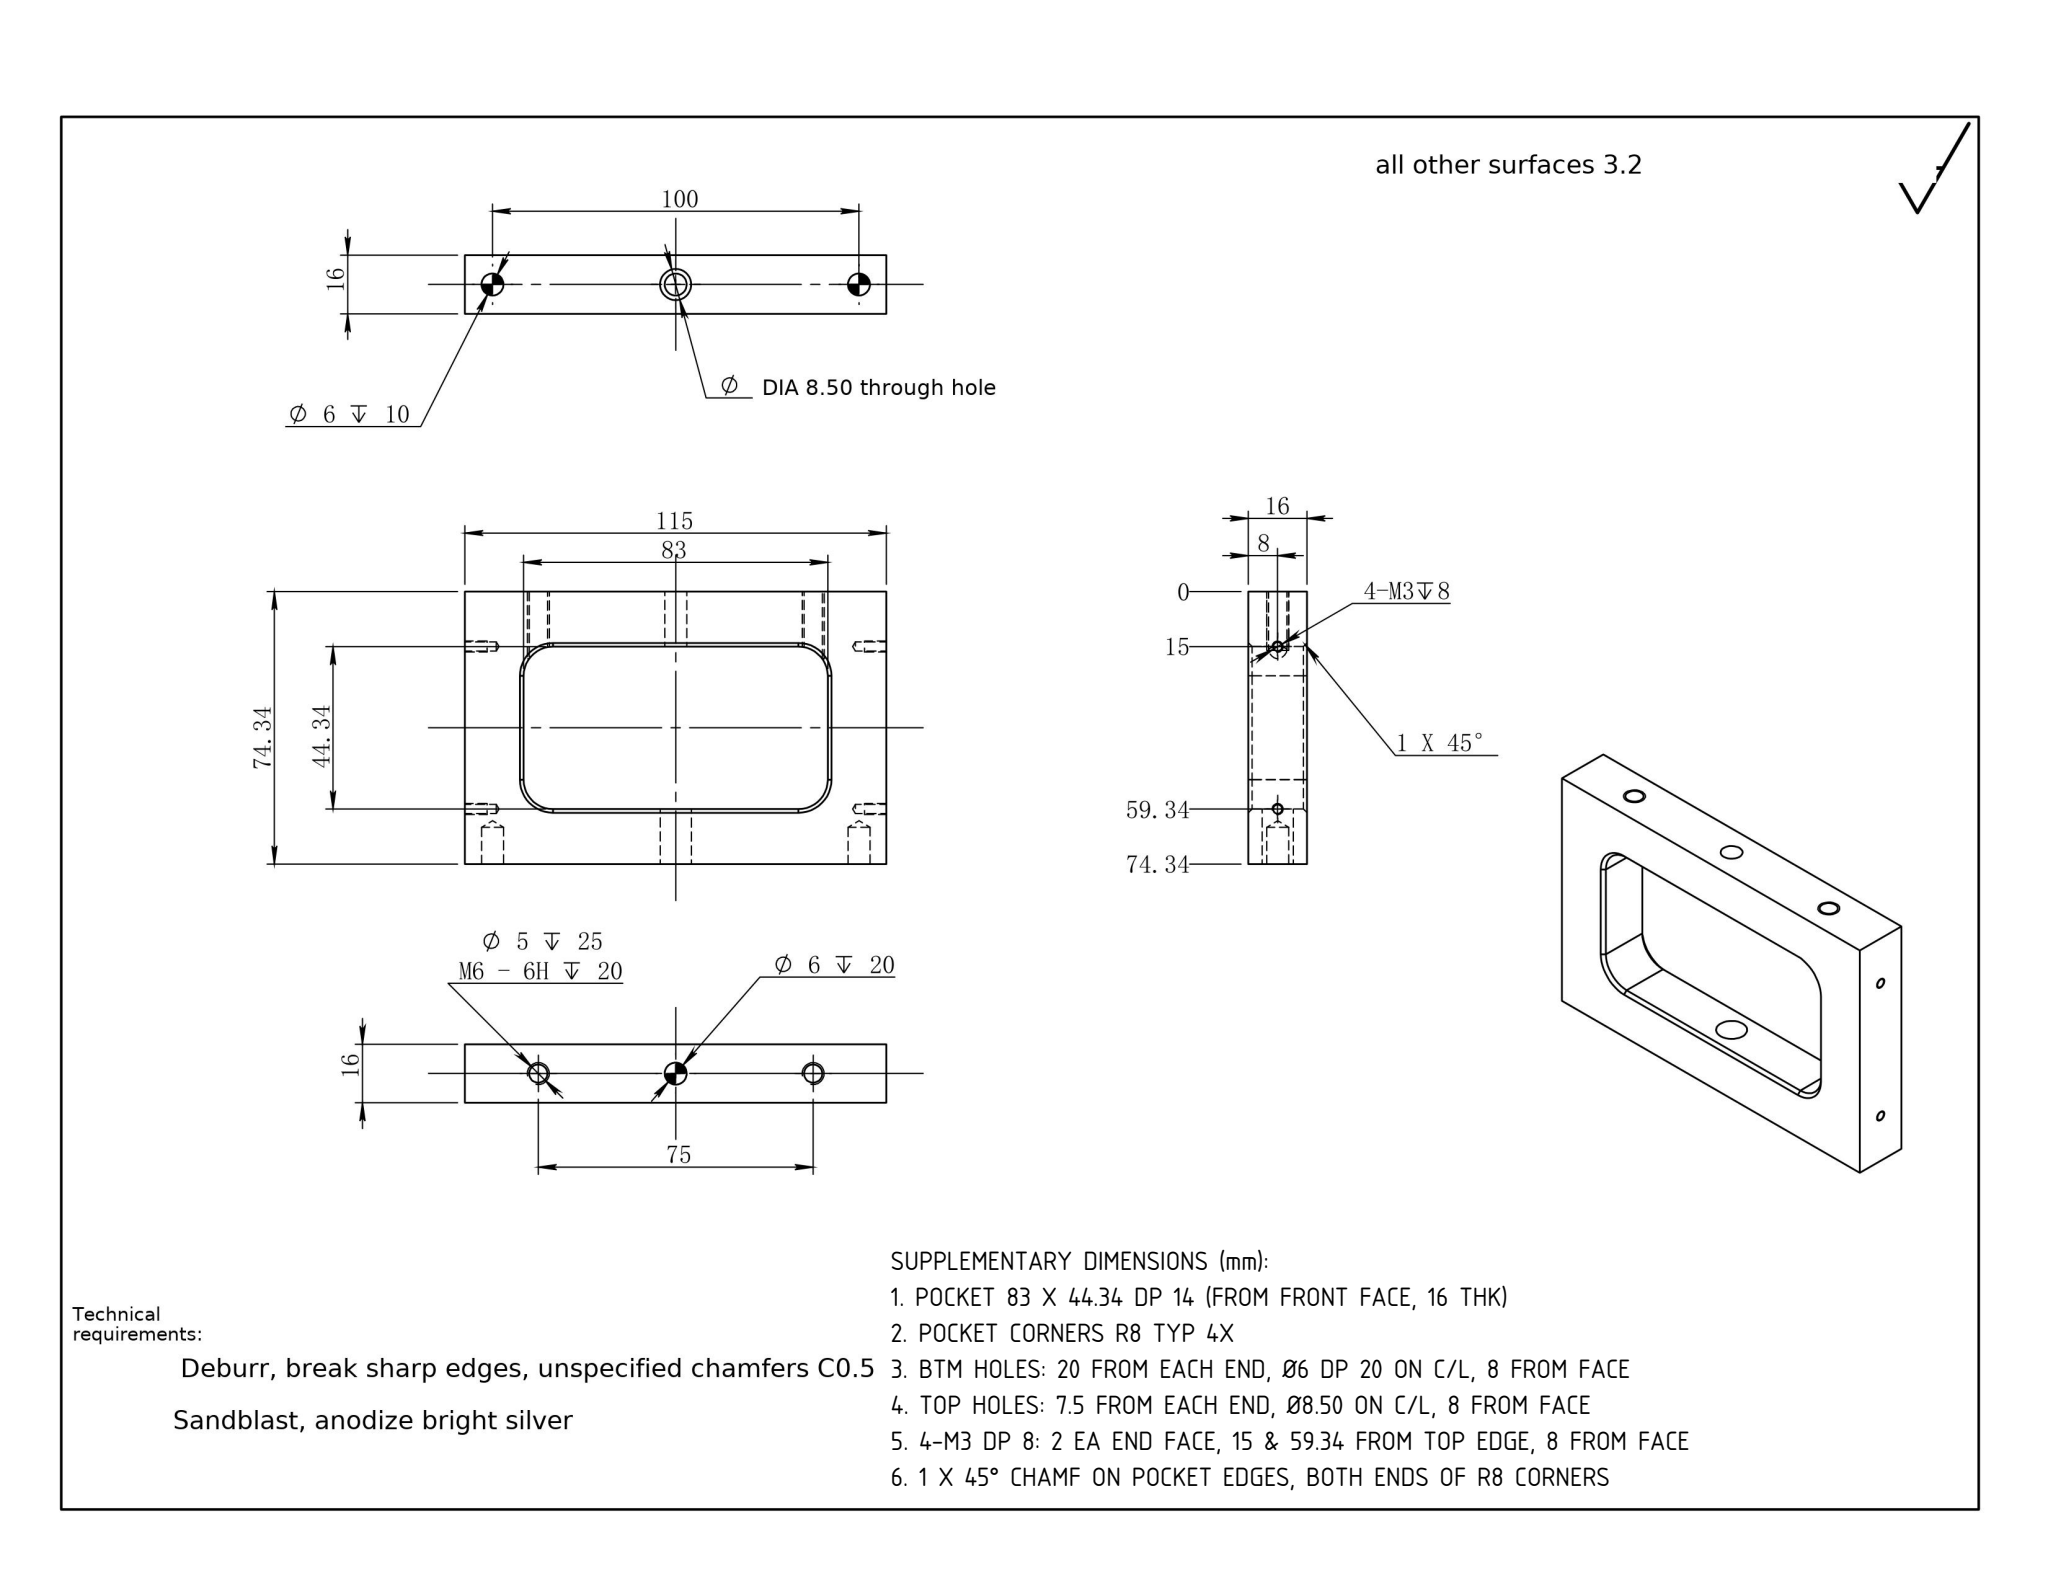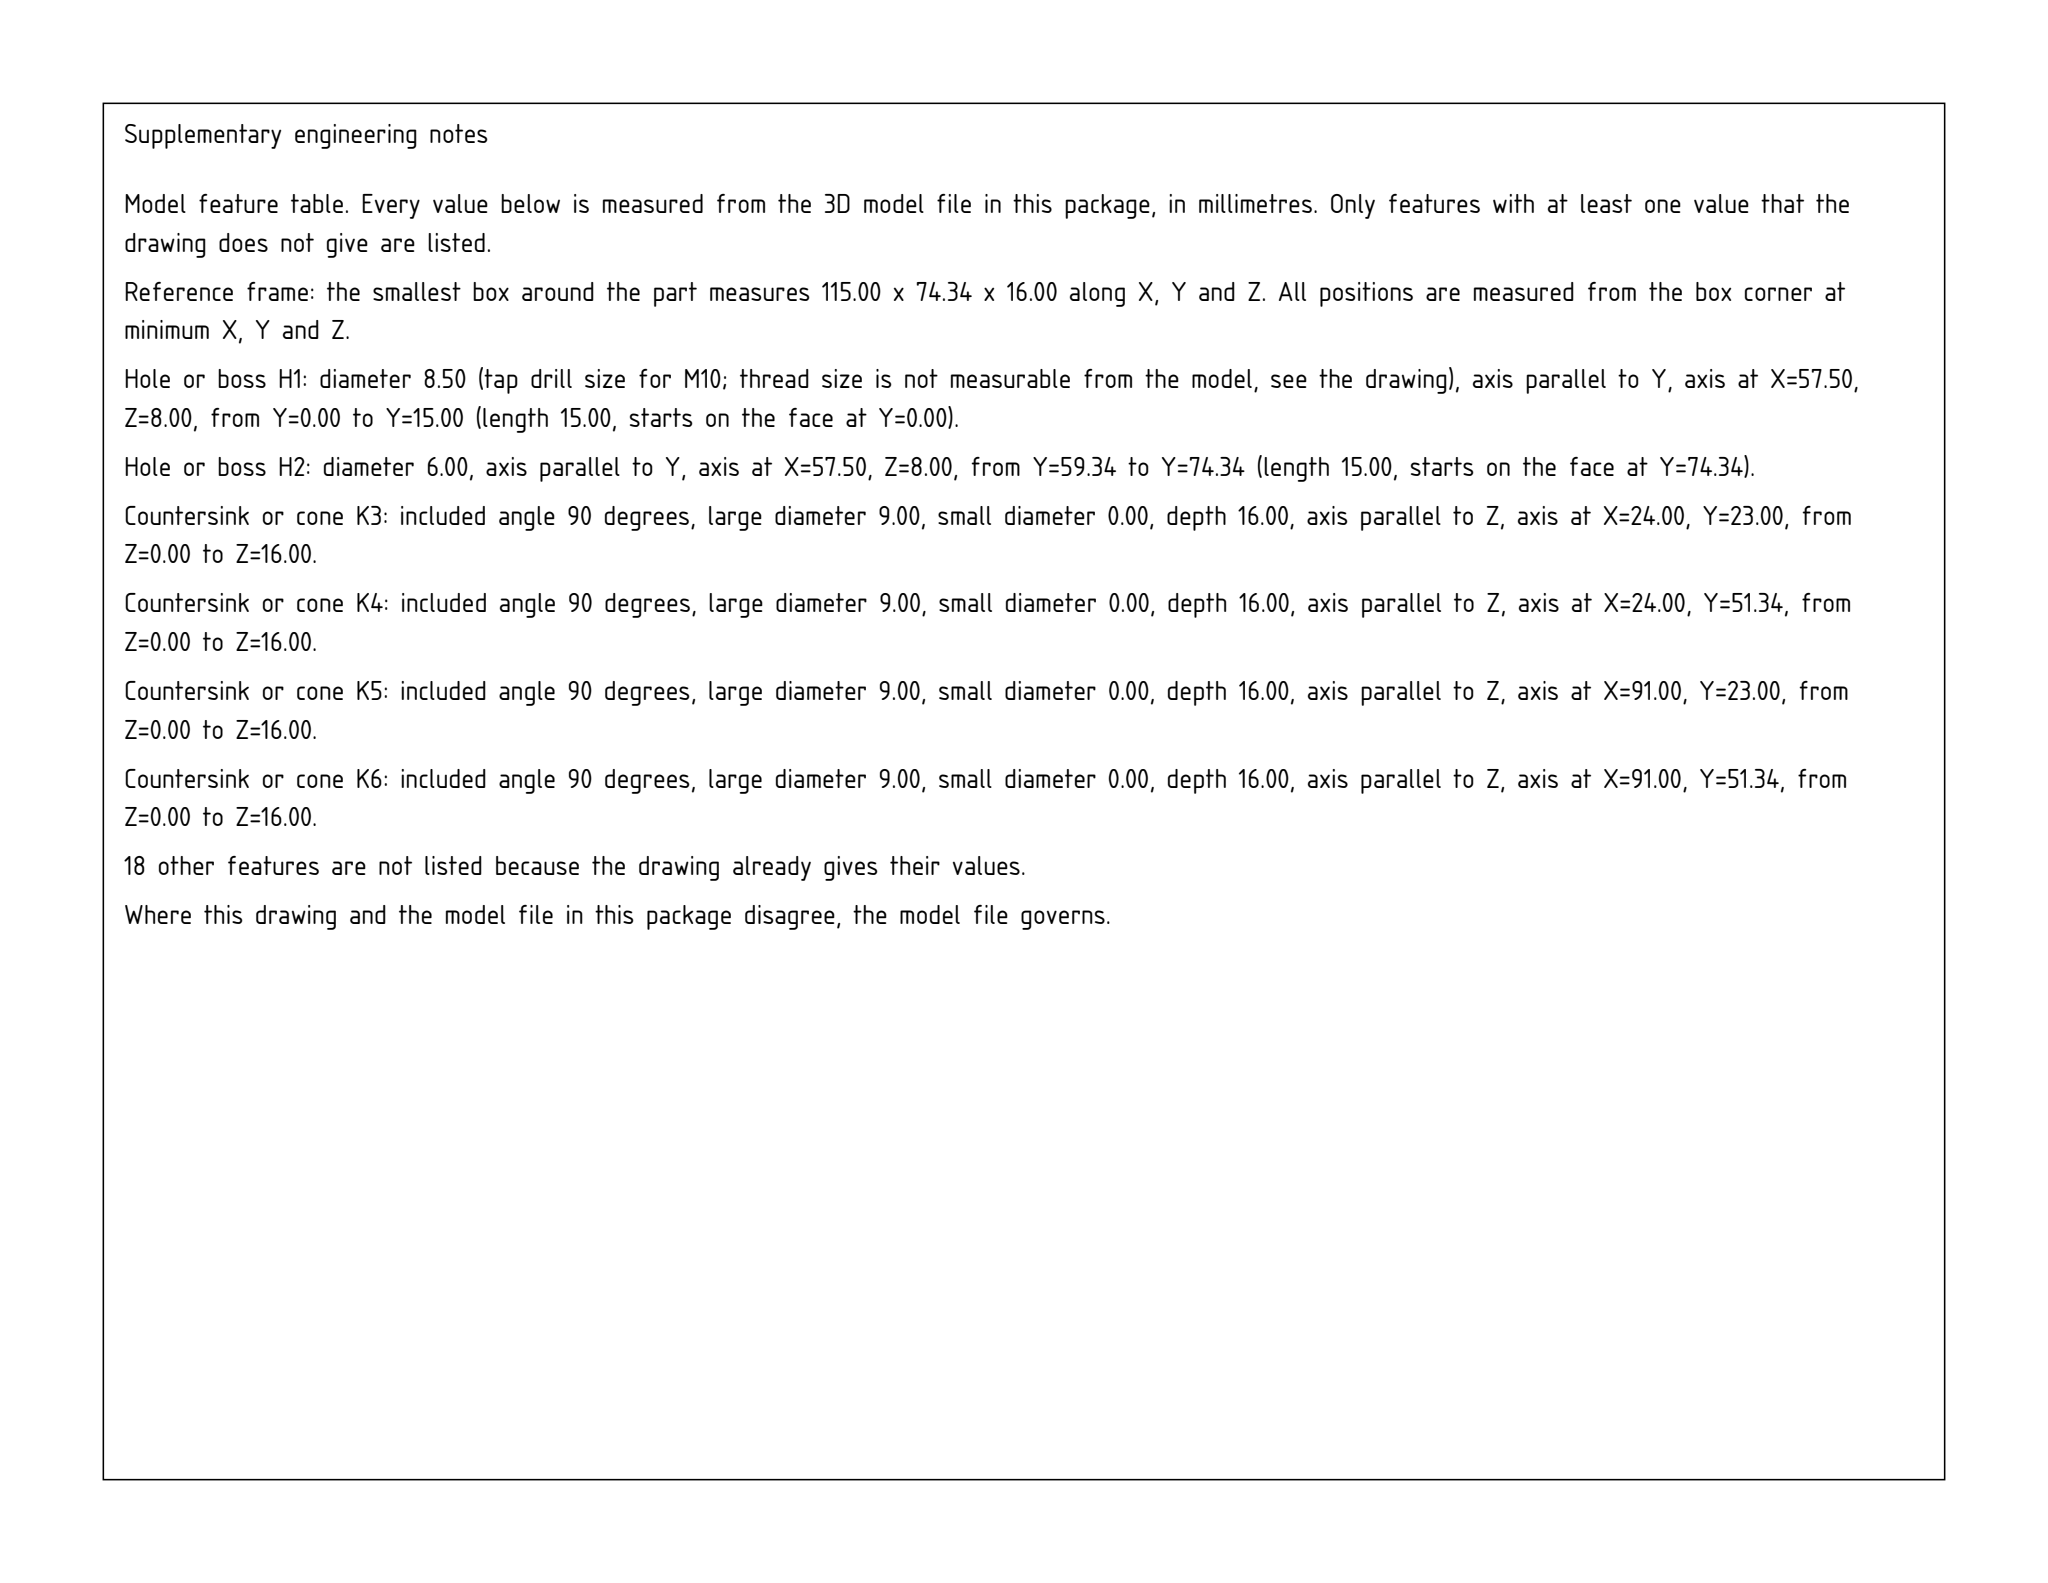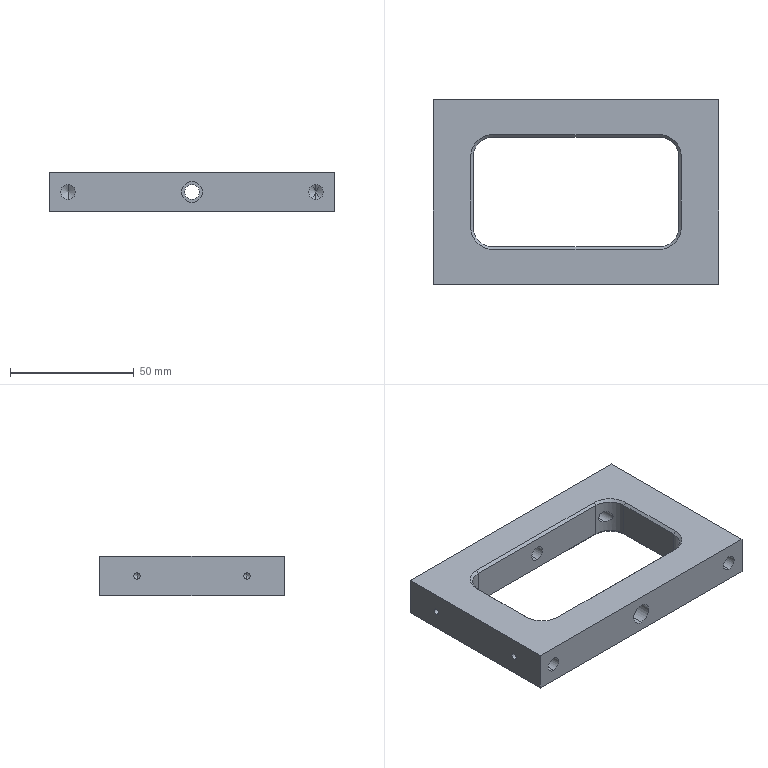Part | SolidWorks | mm | 1 solid | 62 faces | box 115 x 74.34 x 16 mm | volume 75854 mm3 | cylinder 24 | cone 20 | plane 18 | commonest cylinder face diameters 2.5 x8 6 x6 5 x4 16 x4 8.5 x2
build123d program:
from build123d import *

# Parameters (mm, degrees)
SKETCH1_W                      = 115
SKETCH1_H                      = 16
BOSS_EXTRUDE1_DEPTH            = 74.34
SKETCH11_W                     = 83
SKETCH11_H                     = 44.34
CUT_EXTRUDE1_DEPTH             = 96.335
FILLET1_R                      = 8
F_6_0_6_DIAMETER_HOLE2_D       = 6
F_6_0_6_DIAMETER_HOLE2_DEPTH   = 10
F_6_0_6_DIAMETER_HOLE2_TIP     = 1.803
F_6_0_6_DIAMETER_HOLE1_D       = 6
F_6_0_6_DIAMETER_HOLE1_DEPTH   = 20
F_6_0_6_DIAMETER_HOLE1_TIP     = 1.803
M6_TAPPED_HOLE2_D              = 5
M6_TAPPED_HOLE2_DEPTH          = 25
M6_TAPPED_HOLE2_TIP            = 1.502
F_8_5_8_5_DIAMETER_HOLE1_D     = 8.5
F_8_5_8_5_DIAMETER_HOLE1_DEPTH = 15
CHAMFER1_SIZE                  = 1
M3_TAPPED_HOLE1_AT_2_COUNT     = 2
M3_TAPPED_HOLE1_AT_2_PITCH     = 44.34


with BuildPart() as part:
    # Sketch1 → Boss-Extrude1 (new body)
    with BuildSketch(Plane(origin=(0, 0, 0), x_dir=(1, 0, 0), z_dir=(0, 1, 0))):
        Rectangle(SKETCH1_W, SKETCH1_H)
    extrude(amount=BOSS_EXTRUDE1_DEPTH)

    # Sketch11 → Cut-Extrude1 (cut, through all)
    with BuildSketch(Plane.XY.offset(8)):
        with Locations((0, 37.17)):
            Rectangle(SKETCH11_W, SKETCH11_H)
    extrude(amount=-CUT_EXTRUDE1_DEPTH, mode=Mode.SUBTRACT)

    # Fillet1
    fillet1_edges = [part.edges().sort_by_distance(p)[0] for p in [
        (41.5, 59.34, 0),
        (41.5, 15, 0),
        (-41.5, 15, 0),
        (-41.5, 59.34, 0),
    ]]
    fillet(fillet1_edges, radius=FILLET1_R)

    # 6.0 _6_ Diameter Hole2
    with Locations(Plane(origin=(0, 0, 0), x_dir=(-1, 0, 0), z_dir=(0, -1, 0))):
        with Locations((-50, 0), (50, 0)):
            Hole(F_6_0_6_DIAMETER_HOLE2_D / 2, depth=F_6_0_6_DIAMETER_HOLE2_DEPTH)
            with Locations((0, 0, -(F_6_0_6_DIAMETER_HOLE2_DEPTH + F_6_0_6_DIAMETER_HOLE2_TIP / 2))):  # 118° drill point
                Cone(0, F_6_0_6_DIAMETER_HOLE2_D / 2, F_6_0_6_DIAMETER_HOLE2_TIP, mode=Mode.SUBTRACT)

    # 6.0 _6_ Diameter Hole1
    with Locations(Plane(origin=(0, 74.34, 0), x_dir=(-1, 0, 0), z_dir=(0, 1, 0))):
        with Locations((0, 0)):
            Hole(F_6_0_6_DIAMETER_HOLE1_D / 2, depth=F_6_0_6_DIAMETER_HOLE1_DEPTH)
            with Locations((0, 0, -(F_6_0_6_DIAMETER_HOLE1_DEPTH + F_6_0_6_DIAMETER_HOLE1_TIP / 2))):  # 118° drill point
                Cone(0, F_6_0_6_DIAMETER_HOLE1_D / 2, F_6_0_6_DIAMETER_HOLE1_TIP, mode=Mode.SUBTRACT)

    # M6 Tapped Hole2
    with Locations(Plane(origin=(0, 74.34, 0), x_dir=(1, 0, 0), z_dir=(0, 1, 0))):
        with Locations((-37.5, 0), (37.5, 0)):
            Hole(M6_TAPPED_HOLE2_D / 2, depth=M6_TAPPED_HOLE2_DEPTH)
            with Locations((0, 0, -(M6_TAPPED_HOLE2_DEPTH + M6_TAPPED_HOLE2_TIP / 2))):  # 118° drill point
                Cone(0, M6_TAPPED_HOLE2_D / 2, M6_TAPPED_HOLE2_TIP, mode=Mode.SUBTRACT)

    # 8.5 _8.5_ Diameter Hole1
    with Locations(Plane(origin=(0, 15, 0), x_dir=(1, 0, 0), z_dir=(0, 1, 0))):
        with Locations((0, 0)):
            Hole(F_8_5_8_5_DIAMETER_HOLE1_D / 2, depth=F_8_5_8_5_DIAMETER_HOLE1_DEPTH)

    # Chamfer1
    chamfer1_edges = [part.edges().sort_by_distance(p)[0] for p in [
        (41.5, 37.17, 8),
        (41.5, 37.17, -8),
        (0, 15, 8),
        (0, 15, -8),
        (0, 59.34, 8),
        (0, 59.34, -8),
        (-41.5, 37.17, 8),
        (-41.5, 37.17, -8),
        (39.157, 17.343, 8),
        (39.157, 17.343, -8),
        (39.157, 56.997, 8),
        (39.157, 56.997, -8),
        (-39.157, 56.997, 8),
        (-39.157, 56.997, -8),
        (-39.157, 17.343, 8),
        (-39.157, 17.343, -8),
    ]]
    chamfer(chamfer1_edges, length=CHAMFER1_SIZE)

    # Sketch15 → M3 Tapped Hole1 (revolve, cut)
    with BuildSketch(Plane(origin=(57.5, 59.34, 0), x_dir=(0, 0, -1), z_dir=(0, 1, 0))):
        Polygon((0, 0), (0, 9.251), (1.25, 8.5), (1.25, 0), align=None)
    m3_tapped_hole1 = revolve(axis=Axis((63.85, 59.34, 0), (-1, 0, 0)), mode=Mode.SUBTRACT)

    # M3 Tapped Hole1 at 2: M3 Tapped Hole1 ×2
    with Locations(*[(0, -i * M3_TAPPED_HOLE1_AT_2_PITCH, 0) for i in range(1, M3_TAPPED_HOLE1_AT_2_COUNT)]):
        add(m3_tapped_hole1, mode=Mode.SUBTRACT)

    # Mirror1: M3 Tapped Hole1 across plane
    add(m3_tapped_hole1.mirror(Plane(origin=(0, 0, 0), x_dir=(0, 0, 1), z_dir=(1, 0, 0))), mode=Mode.SUBTRACT)

    # Mirror1 copy 1 sketch → Mirror1 copy 1 (revolve, cut)
    with BuildSketch(Plane(origin=(-57.5, 15, 0), x_dir=(0, 0, -1), z_dir=(0, 1, 0))):
        Polygon((0, 0), (0, -9.251), (1.25, -8.5), (1.25, 0), align=None)
    revolve(axis=Axis((-63.85, 15, 0), (-1, 0, 0)), mode=Mode.SUBTRACT)


solid = part.part